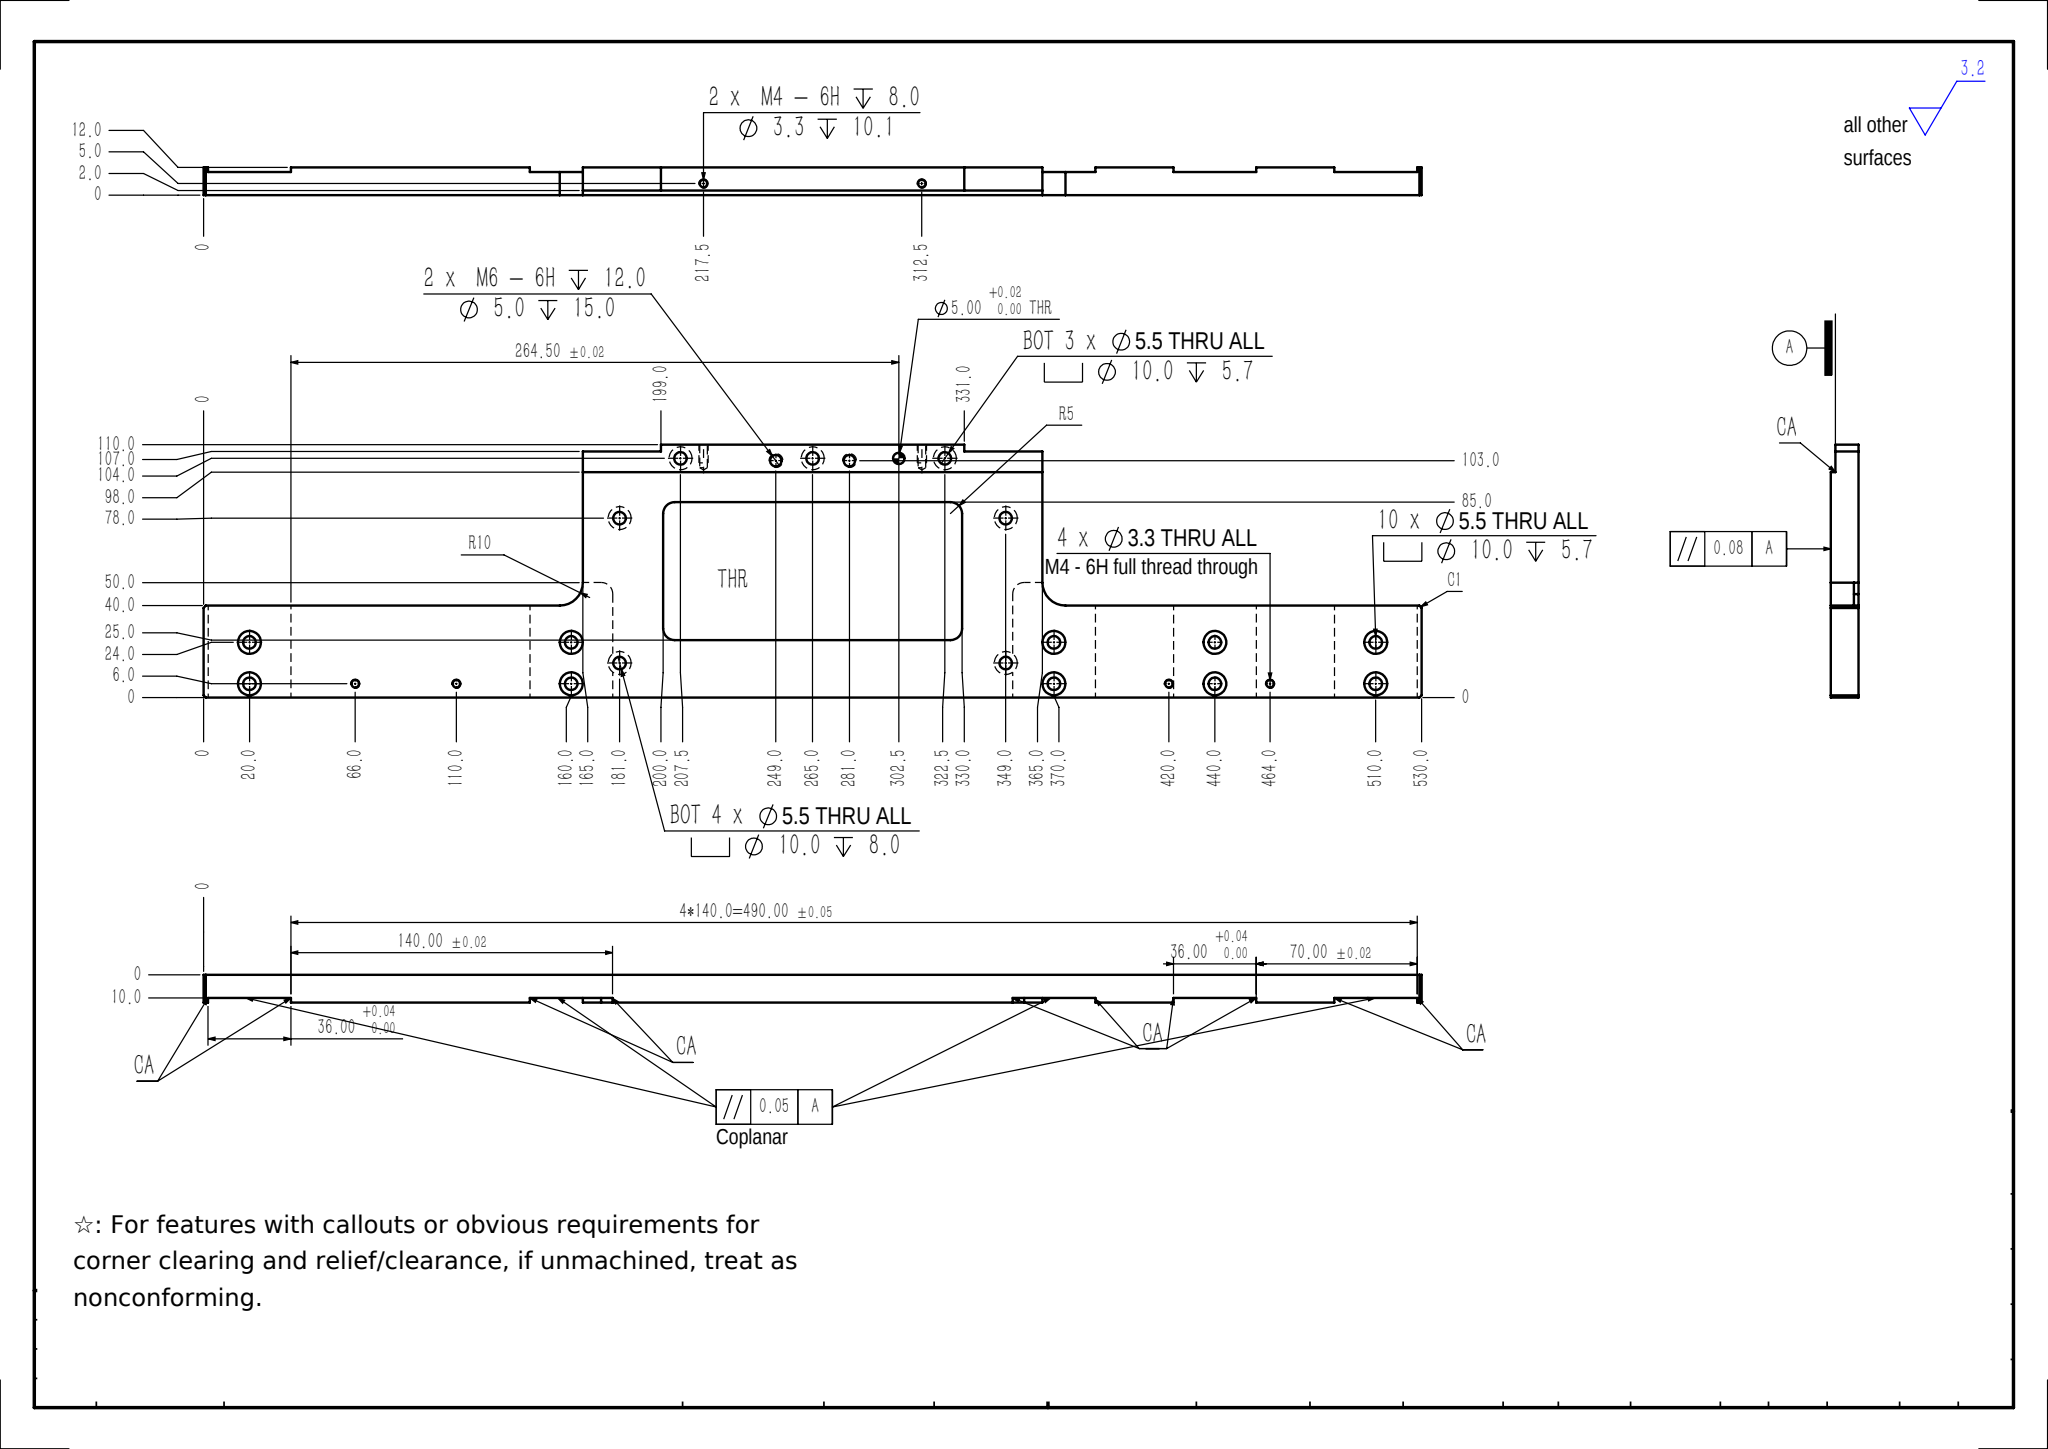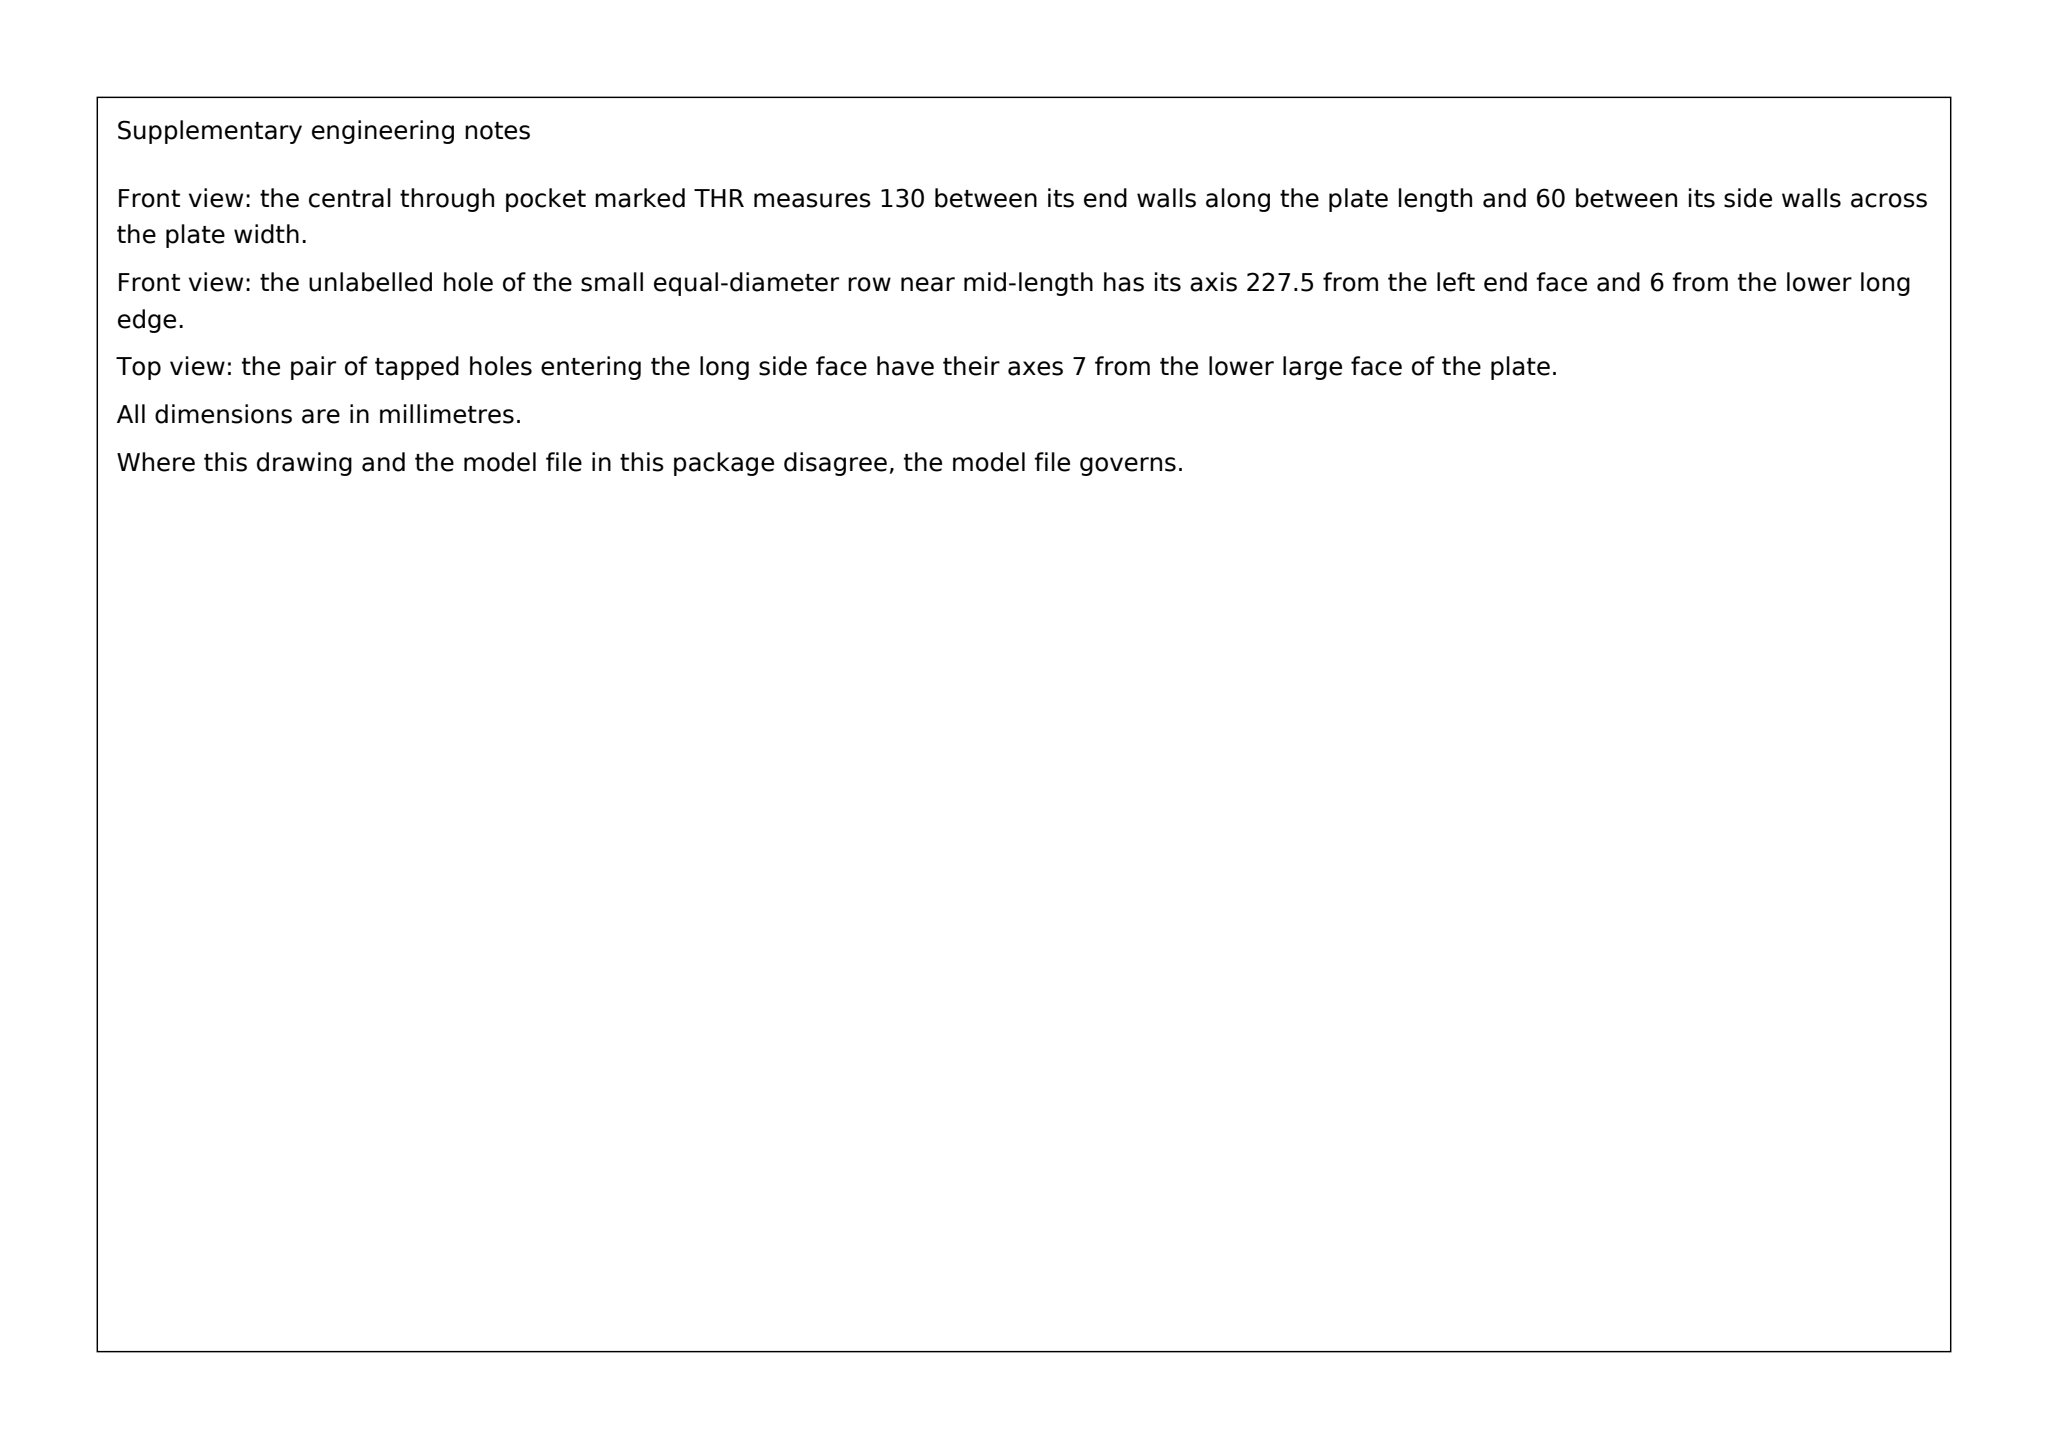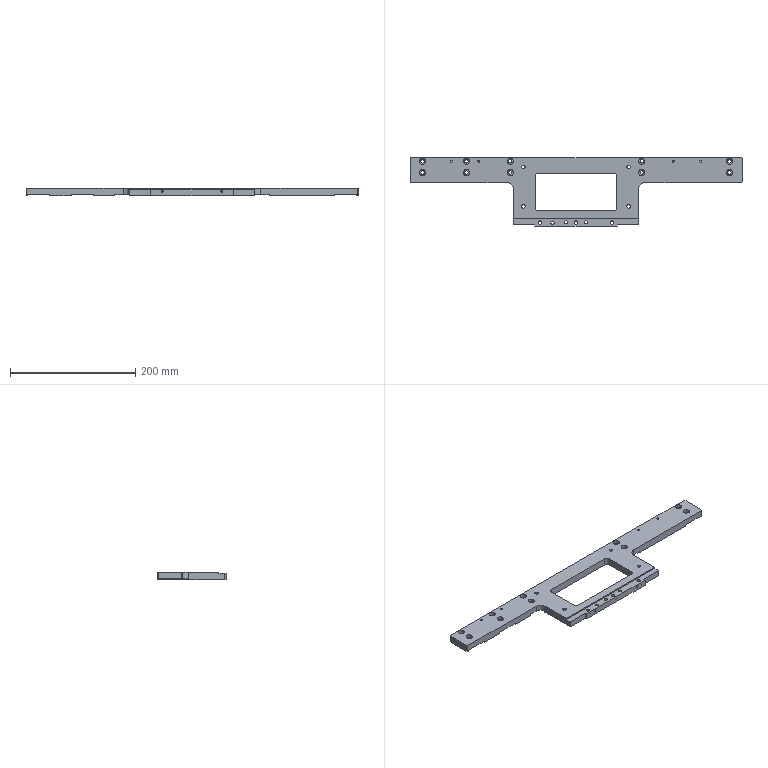Part | SolidWorks | mm | 1 solid | 163 faces | box 530 x 110 x 12 mm | volume 296550 mm3 | cylinder 94 | plane 65 | cone 4 | commonest cylinder face diameters 10 x40 5.5 x34 3.3 x12 5 x6 20 x2
build123d program:
from build123d import *

# Parameters (mm, degrees)
SKETCH1_W                                         = 530
SKETCH1_H                                         = 110
BOSS_EXTRUDE1_DEPTH                               = 12
SKETCH2_W                                         = 165
SKETCH2_H                                         = 70
CUT_EXTRUDE1_DEPTH                                = 271.913
FILLET1_R                                         = 10
SKETCH3_W                                         = 200
SKETCH3_H                                         = 12
CUT_EXTRUDE2_DEPTH                                = 2
SKETCH4_W                                         = 34
SKETCH4_H                                         = 3
CUT_EXTRUDE3_DEPTH                                = 271.913
SKETCH5_W                                         = 36
SKETCH5_H                                         = 40
SKETCH5_H_2                                       = 50
CUT_EXTRUDE4_DEPTH                                = 2
FILLET2_R                                         = 5
M6_TAPPED_HOLE1_D                                 = 5
M6_TAPPED_HOLE1_DEPTH                             = 15
M6_TAPPED_HOLE1_TIP                               = 1.502
HOLE_SIZE_ACCORDING_TO_TYPE_OF_HEXAGO_D           = 5.5
HOLE_SIZE_ACCORDING_TO_TYPE_OF_HEXAGO_CBORE_D     = 10
HOLE_SIZE_ACCORDING_TO_TYPE_OF_HEXAGO_CBORE_DEPTH = 5.7
HOLE_SIZE_ACCORDING_TO_TYPE_OF_HE_2_D             = 5.5
HOLE_SIZE_ACCORDING_TO_TYPE_OF_HE_2_CBORE_D       = 10
HOLE_SIZE_ACCORDING_TO_TYPE_OF_HE_2_CBORE_DEPTH   = 8
HOLE_SIZE_ACCORDING_TO_TYPE_OF_HE_3_D             = 5.5
HOLE_SIZE_ACCORDING_TO_TYPE_OF_HE_3_CBORE_D       = 10
HOLE_SIZE_ACCORDING_TO_TYPE_OF_HE_3_CBORE_DEPTH   = 5.7
SIZE_MM_DOWEL_PIN_HOLE1_D                         = 5
SKETCH17_W                                        = 130
SKETCH17_H                                        = 60
CUT_EXTRUDE6_DEPTH                                = 271.913
FILLET3_R                                         = 5
M4_TAPPED_HOLE1_D                                 = 3.3
M4_TAPPED_HOLE1_DEPTH                             = 10.1
M4_TAPPED_HOLE1_TIP                               = 0.9914
CHAMFER1_SIZE                                     = 1
M4_TAPPED_HOLE2_D                                 = 3.3


with BuildPart() as part:
    # Sketch1 → Boss-Extrude1 (new body)
    with BuildSketch(Plane.XY):
        Rectangle(SKETCH1_W, SKETCH1_H)
    extrude(amount=BOSS_EXTRUDE1_DEPTH)

    # Sketch2 → Cut-Extrude1 (cut, through all)
    with BuildSketch(Plane.XY.offset(12)):
        with Locations((-182.5, -20)):
            Rectangle(SKETCH2_W, SKETCH2_H)
        with Locations((182.5, -20)):
            Rectangle(SKETCH2_W, SKETCH2_H)
    extrude(amount=-CUT_EXTRUDE1_DEPTH, mode=Mode.SUBTRACT)

    # Fillet1
    fillet1_edges = [part.edges().sort_by_distance(p)[0] for p in [
        (-100, 15, 6),
        (100, 15, 6),
    ]]
    fillet(fillet1_edges, radius=FILLET1_R)

    # Sketch3 → Cut-Extrude2 (cut)
    with BuildSketch(Plane.XY.offset(12)):
        with Locations((0, -49)):
            Rectangle(SKETCH3_W, SKETCH3_H)
    extrude(amount=-CUT_EXTRUDE2_DEPTH, mode=Mode.SUBTRACT)

    # Sketch4 → Cut-Extrude3 (cut, through all)
    with BuildSketch(Plane.XY.offset(12)):
        with Locations((83, -53.5)):
            Rectangle(SKETCH4_W, SKETCH4_H)
        with Locations((-83, -53.5)):
            Rectangle(SKETCH4_W, SKETCH4_H)
    extrude(amount=-CUT_EXTRUDE3_DEPTH, mode=Mode.SUBTRACT)

    # Sketch5 → Cut-Extrude4 (cut)
    with BuildSketch(Plane(origin=(0, 0, 0), x_dir=(-1, 0, 0), z_dir=(0, 0, -1))):
        with Locations((245, 35)):
            Rectangle(SKETCH5_W, SKETCH5_H)
        with Locations((105, 30)):
            Rectangle(SKETCH5_W, SKETCH5_H_2)
        with Locations((-105, 30)):
            Rectangle(SKETCH5_W, SKETCH5_H_2)
        with Locations((-245, 35)):
            Rectangle(SKETCH5_W, SKETCH5_H)
        with Locations((175, 35)):
            Rectangle(SKETCH5_W, SKETCH5_H)
    extrude(amount=-CUT_EXTRUDE4_DEPTH, mode=Mode.SUBTRACT)

    # Fillet2
    fillet2_edges = [part.edges().sort_by_distance(p)[0] for p in [
        (87, 5, 1),
        (-87, 5, 1),
    ]]
    fillet(fillet2_edges, radius=FILLET2_R)

    # M6 Tapped Hole1
    with Locations(Plane(origin=(0, 0, 0), x_dir=(-1, 0, 0), z_dir=(0, 0, -1))):
        with Locations((-16, -48), (16, -48)):
            Hole(M6_TAPPED_HOLE1_D / 2, depth=M6_TAPPED_HOLE1_DEPTH)
            with Locations((0, 0, -(M6_TAPPED_HOLE1_DEPTH + M6_TAPPED_HOLE1_TIP / 2))):  # 118° drill point
                Cone(0, M6_TAPPED_HOLE1_D / 2, M6_TAPPED_HOLE1_TIP, mode=Mode.SUBTRACT)

    # Hole Size _ according to_ type of Hexago (through all)
    with Locations(Plane.XY.offset(12)):
        with Locations((-105, 31), (-105, 49), (105, 31), (105, 49), (245, 31), (245, 49), (-245, 31), (-245, 49), (-175, 49), (-175, 31)):
            CounterBoreHole(HOLE_SIZE_ACCORDING_TO_TYPE_OF_HEXAGO_D / 2, HOLE_SIZE_ACCORDING_TO_TYPE_OF_HEXAGO_CBORE_D / 2, HOLE_SIZE_ACCORDING_TO_TYPE_OF_HEXAGO_CBORE_DEPTH)

    # Hole Size _ according to_ type of He 2 (through all)
    with Locations(Plane(origin=(0, 0, 0), x_dir=(-1, 0, 0), z_dir=(0, 0, -1))):
        with Locations((-84, 40), (-84, -23), (84, 40), (84, -23)):
            CounterBoreHole(HOLE_SIZE_ACCORDING_TO_TYPE_OF_HE_2_D / 2, HOLE_SIZE_ACCORDING_TO_TYPE_OF_HE_2_CBORE_D / 2, HOLE_SIZE_ACCORDING_TO_TYPE_OF_HE_2_CBORE_DEPTH)

    # Hole Size _ according to_ type of He 3 (through all)
    with Locations(Plane(origin=(0, 0, 0), x_dir=(-1, 0, 0), z_dir=(0, 0, -1))):
        with Locations((57.5, -49), (0, -49), (-57.5, -49)):
            CounterBoreHole(HOLE_SIZE_ACCORDING_TO_TYPE_OF_HE_3_D / 2, HOLE_SIZE_ACCORDING_TO_TYPE_OF_HE_3_CBORE_D / 2, HOLE_SIZE_ACCORDING_TO_TYPE_OF_HE_3_CBORE_DEPTH)

    # Size mm Dowel Pin Hole1 (through all)
    with Locations(Plane(origin=(0, 0, 0), x_dir=(-1, 0, 0), z_dir=(0, 0, -1))):
        with Locations((37.5, -49)):
            Hole(SIZE_MM_DOWEL_PIN_HOLE1_D / 2)

    # Sketch17 → Cut-Extrude6 (cut, through all)
    with BuildSketch(Plane(origin=(0, 0, 0), x_dir=(-1, 0, 0), z_dir=(0, 0, -1))):
        Rectangle(SKETCH17_W, SKETCH17_H)
    extrude(amount=-CUT_EXTRUDE6_DEPTH, mode=Mode.SUBTRACT)

    # Fillet3
    fillet3_edges = [part.edges().sort_by_distance(p)[0] for p in [
        (-65, 30, 6),
        (-65, -30, 6),
        (65, -30, 6),
        (65, 30, 6),
    ]]
    fillet(fillet3_edges, radius=FILLET3_R)

    # M4 Tapped Hole1
    with Locations(Plane(origin=(0, -55, 0), x_dir=(-1, 0, 0), z_dir=(0, -1, 0))):
        with Locations((47.5, -7), (-47.5, -7)):
            Hole(M4_TAPPED_HOLE1_D / 2, depth=M4_TAPPED_HOLE1_DEPTH)
            with Locations((0, 0, -(M4_TAPPED_HOLE1_DEPTH + M4_TAPPED_HOLE1_TIP / 2))):  # 118° drill point
                Cone(0, M4_TAPPED_HOLE1_D / 2, M4_TAPPED_HOLE1_TIP, mode=Mode.SUBTRACT)

    # Chamfer1
    chamfer1_edges = [part.edges().sort_by_distance(p)[0] for p in [
        (-265, 15, 6),
        (265, 15, 6),
        (-265, 55, 6),
        (265, 55, 6),
    ]]
    chamfer(chamfer1_edges, length=CHAMFER1_SIZE)

    # M4 Tapped Hole2 (through all)
    with Locations(Plane.XY.offset(12)):
        with Locations((199, 49), (155, 49), (-155, 49), (-199, 49)):
            Hole(M4_TAPPED_HOLE2_D / 2)


solid = part.part